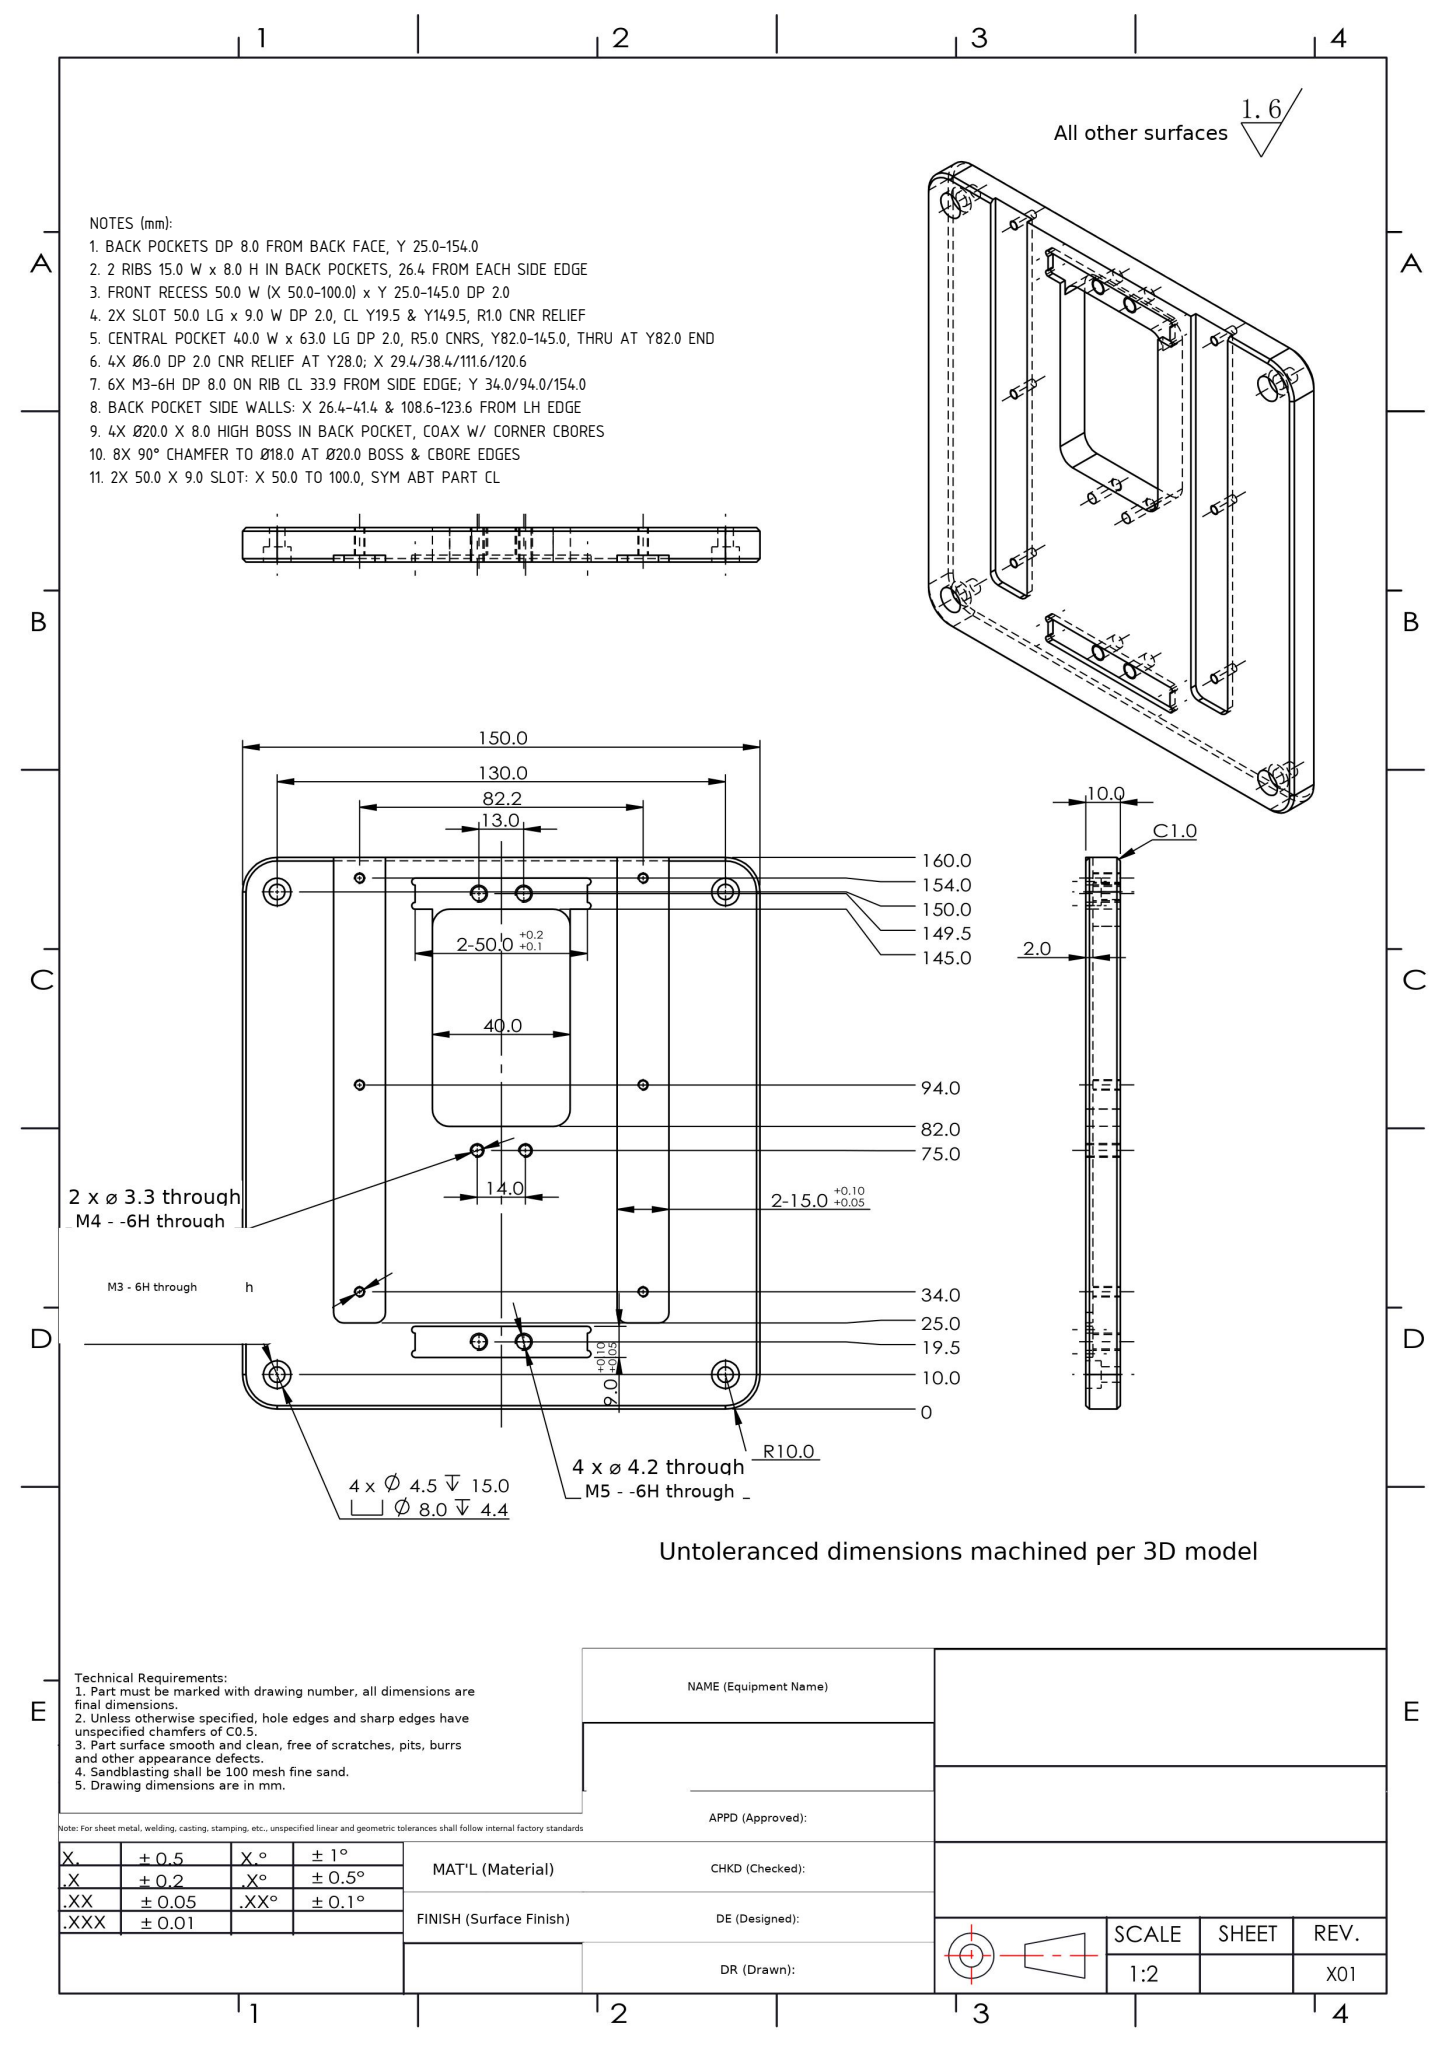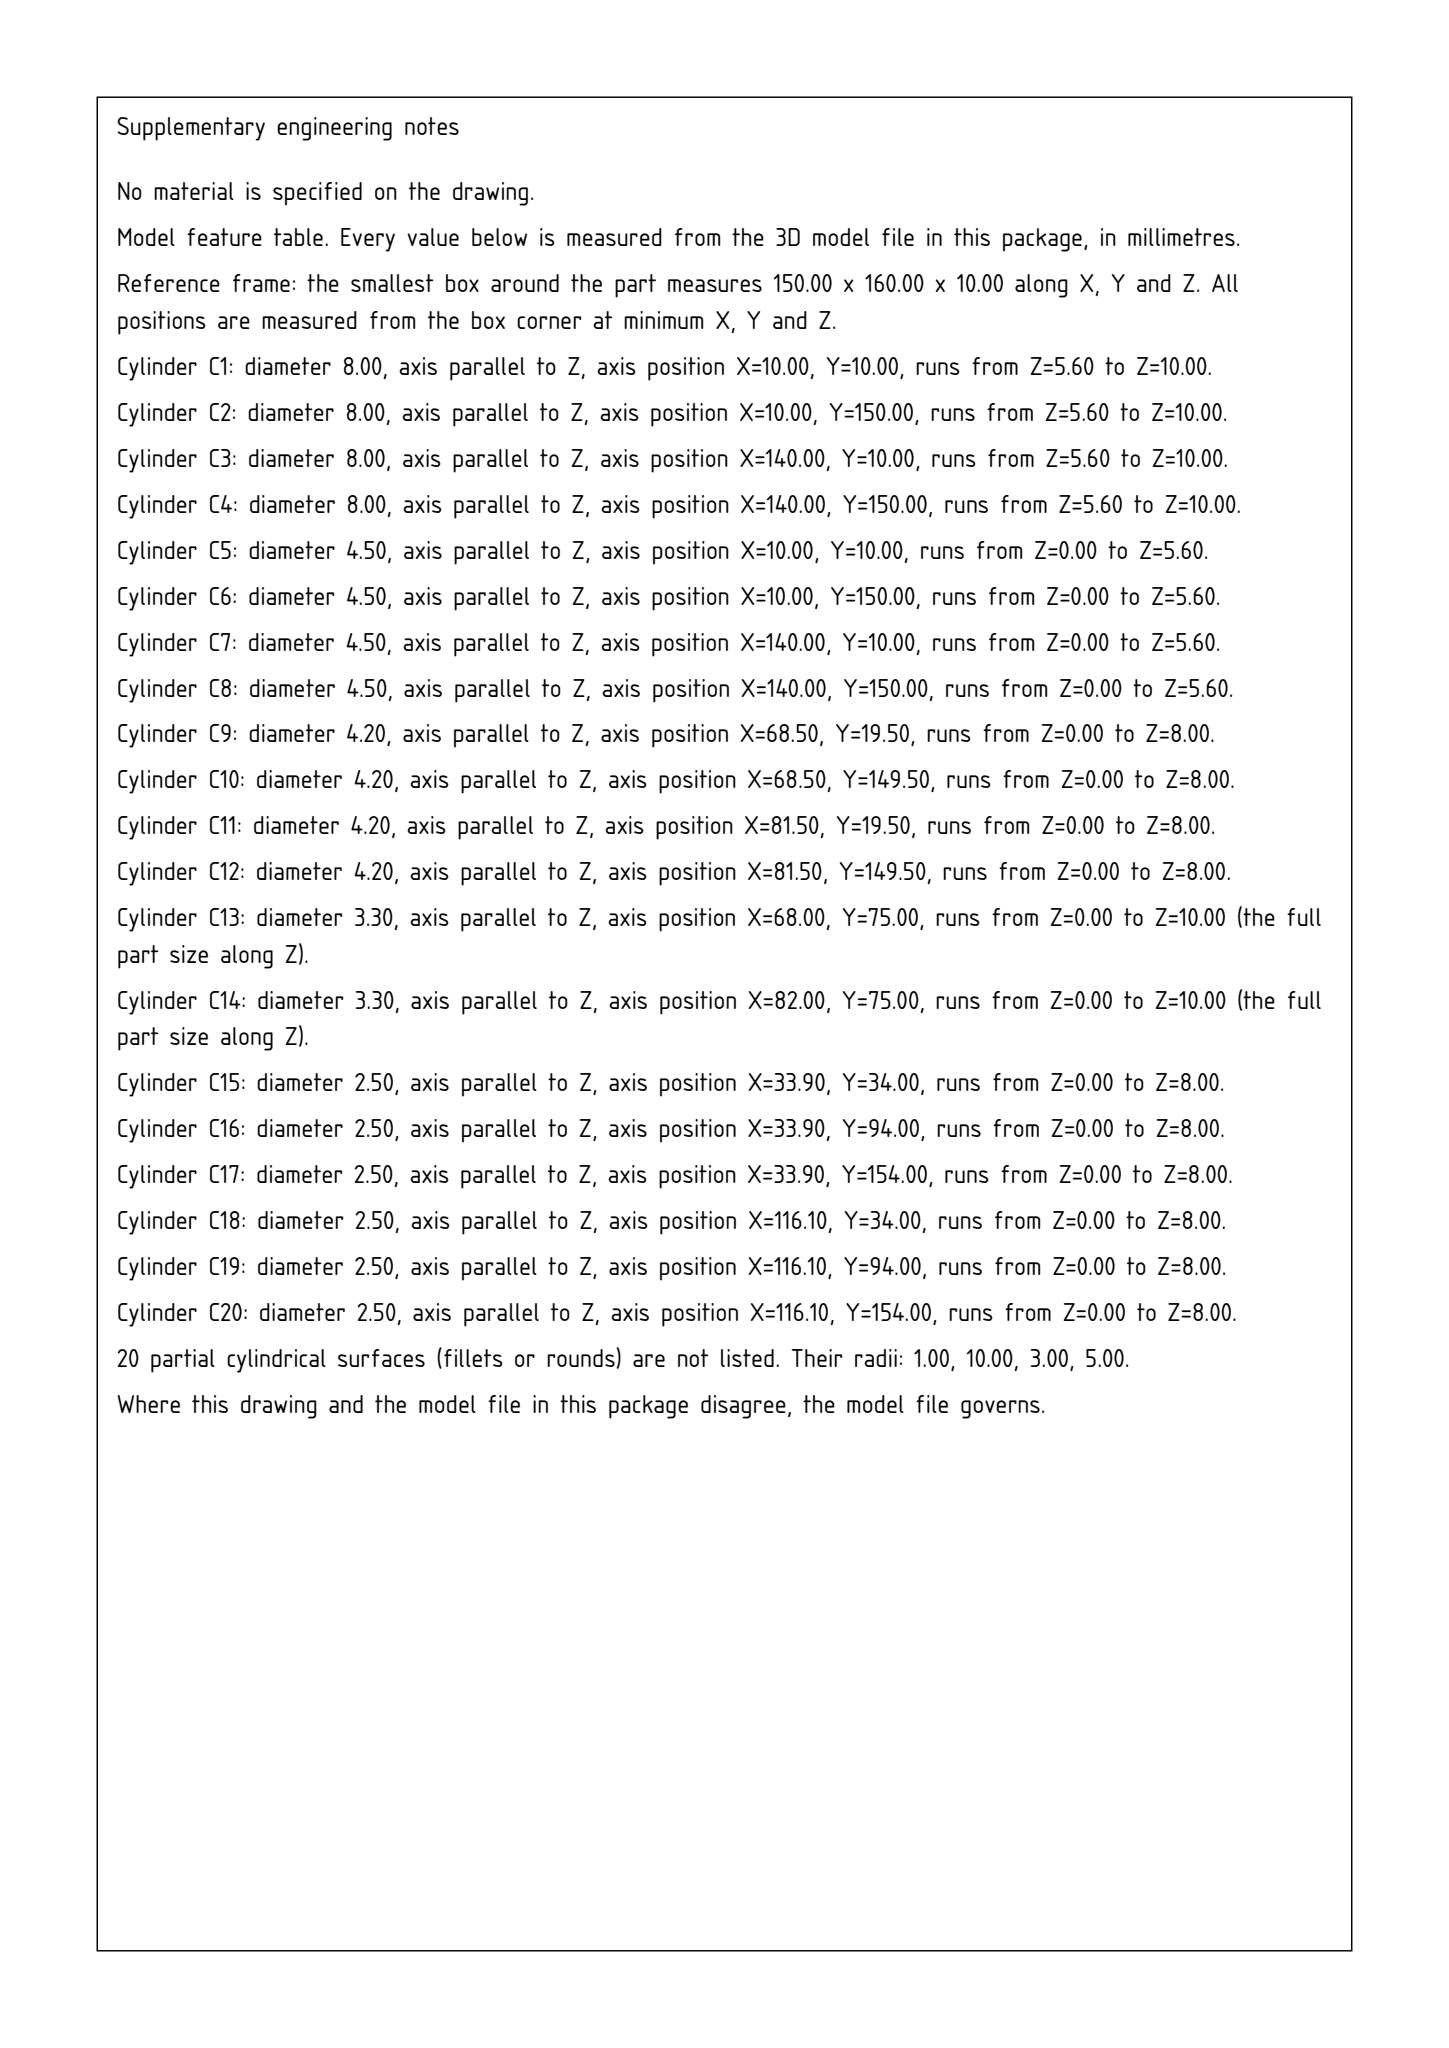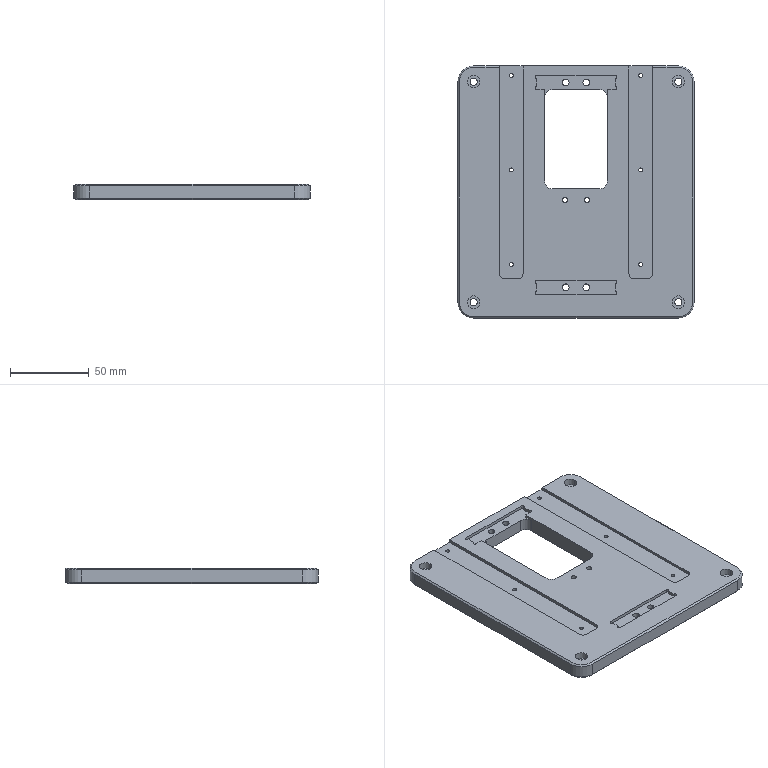Part | SolidWorks | mm | 1 solid | 114 faces | box 150 x 160 x 10 mm | volume 201582 mm3 | cylinder 64 | plane 42 | cone 8 | commonest cylinder face diameters 2 x12 2.5 x12 4.2 x8 8 x8 4.5 x8 3.3 x4 6 x4 20 x4
Drawing notes:
BACK POCKETS DP 8.0 FROM BACK FACE, Y 25.0-154.0 | from the solid: z-planes 0/8.0 (4 faces)/10.0 -> 8.0 dp pockets, 2.0 web; y-planes 25.0 (2x) and 154.0
2 RIBS 15.0 W x 8.0 H IN BACK POCKETS, 26.4 FROM EACH SIDE EDGE | from the solid: x-planes 26.4/41.4 and 108.6/123.6 = 15.0 W ribs, 26.4 from x=0 and x=150; rib top z=8.0
FRONT RECESS 50.0 W (X 50.0-100.0) x Y 25.0-145.0 DP 2.0 | from the solid: x-planes 50.0 & 100.0, y-planes 25.0 & 145.0, floor z=8.0 below front face z=10.0
2X SLOT 50.0 LG x 9.0 W DP 2.0, CL Y19.5 & Y149.5, R1.0 CNR RELIEF | from the solid: y 15.0/24.0 and 145.0/154.0 = 9.0 W, CL 19.5/149.5; x 50.0-100.0; O2.0 x 2.0 lg cyls at (50,16)(50,23)(100,16)(100,23)
CENTRAL POCKET 40.0 W x 63.0 LG DP 2.0, R5.0 CNRS, Y82.0-145.0, THRU AT Y82.0 END | from the solid: planes x55.0/95.0, y82.0/145.0; O10.0 cyls len 8.0 at (60,140)(90,140) and len 10.0 (thru) at (60,87)(90,87)
4X Ø6.0 DP 2.0 CNR RELIEF AT Y28.0; X 29.4/38.4/111.6/120.6 | from the solid: O6.0 z-cyls len 2.0 at (29.4,28),(38.4,28),(111.6,28),(120.6,28)
6X M3-6H DP 8.0 ON RIB CL 33.9 FROM SIDE EDGE; Y 34.0/94.0/154.0 | from the solid: O2.5 x 8.0 lg holes at x=33.9 & 116.1 (rib CL), y=34.0, 94.0, 154.0
BACK POCKET SIDE WALLS: X 26.4-41.4 & 108.6-123.6 FROM LH EDGE | from the solid: axis_planes x = 26.4, 41.4, 108.6, 123.6 (each 15.0 wide, CL 33.9/116.1 = M3 hole CL), pocket Y 25.0-154.0, DP 8.0 (z plane 8.0 x4)
4X Ø20.0 X 8.0 HIGH BOSS IN BACK POCKET, COAX W/ CORNER CBORES | from the solid: cylinders [20.0, z, (10,10)(10,150)(140,10)(140,150), L=8.0] coaxial with Ø4.5/Ø8.0 corner holes
8X 90° CHAMFER TO Ø18.0 AT Ø20.0 BOSS & CBORE EDGES | from the solid: cones [included_angle 90.0, ref_dia 18.0] count 8
2X 50.0 X 9.0 SLOT: X 50.0 TO 100.0, SYM ABT PART CL | from the solid: axis_planes x=50.0 (2), x=100.0 (2); y=15.0/24.0 and y=145.0/154.0 give 9.0 width at CL 19.5 & 149.5; bbox X 150.0 so CL = 75.0
build123d program:
from build123d import *

# Parameters (mm, degrees)
BOSS_EXTRUDE1_DEPTH                             = 10
CUT_EXTRUDE1_DEPTH                              = 111.114
M4_HEX_SOCKET_HEAD_CAP_SCREW_CBORE1_D           = 4.5
M4_HEX_SOCKET_HEAD_CAP_SCREW_CBORE1_DEPTH       = 15
M4_HEX_SOCKET_HEAD_CAP_SCREW_CBORE1_CBORE_D     = 8
M4_HEX_SOCKET_HEAD_CAP_SCREW_CBORE1_CBORE_DEPTH = 4.4
M4_HEX_SOCKET_HEAD_CAP_SCREW_CBORE1_TIP         = 1.352
CUT_EXTRUDE2_DEPTH                              = 2
FILLET1_R                                       = 3
M3_TAPPED_HOLE1_D                               = 2.5
FILLET2_R                                       = 10
FILLET3_R                                       = 5
SKETCH10_W                                      = 50
SKETCH10_H                                      = 9
SKETCH10_H_2                                    = 9
CUT_EXTRUDE3_DEPTH                              = 2
SKETCH11_W                                      = 5
SKETCH11_H                                      = 5
CUT_EXTRUDE4_DEPTH                              = 2
HOLE1_AT_2_COUNT                                = 2
HOLE1_AT_2_PITCH                                = 7
HOLE1_AT_3_COUNT                                = 2
HOLE1_AT_3_PITCH                                = 50.488
HOLE1_AT_4_COUNT                                = 2
HOLE1_AT_4_PITCH                                = 50
HOLE1_AT_5_COUNT                                = 2
HOLE1_AT_5_PITCH                                = 139.284
HOLE1_AT_6_COUNT                                = 2
HOLE1_AT_6_PITCH                                = 145.839
HOLE1_AT_7_COUNT                                = 2
HOLE1_AT_7_PITCH                                = 137
HOLE1_AT_8_COUNT                                = 2
HOLE1_AT_8_PITCH                                = 130
M5_TAPPED_HOLE2_D                               = 4.2
CHAMFER1_SIZE                                   = 1
M4_TAPPED_HOLE1_D                               = 3.3


with BuildPart() as part:
    # Sketch1 → Boss-Extrude1 (new body)
    with BuildSketch(Plane.XY):
        Polygon((75, -80), (-75, -80), (-75, 80), (75, 80), align=None)
    extrude(amount=BOSS_EXTRUDE1_DEPTH)

    # Sketch2 → Cut-Extrude1 (cut, through all)
    with BuildSketch(Plane(origin=(0, 0, 0), x_dir=(-1, 0, 0), z_dir=(0, 0, -1))):
        Polygon((20, 65), (-20, 65), (-20, 2), (20, 2), align=None)
    extrude(amount=-CUT_EXTRUDE1_DEPTH, mode=Mode.SUBTRACT)

    # M4 Hex Socket Head Cap Screw CBORE1
    with Locations(Plane.XY.offset(10)):
        with Locations((-65, -70), (65, -70), (65, 70), (-65, 70)):
            CounterBoreHole(M4_HEX_SOCKET_HEAD_CAP_SCREW_CBORE1_D / 2, M4_HEX_SOCKET_HEAD_CAP_SCREW_CBORE1_CBORE_D / 2, M4_HEX_SOCKET_HEAD_CAP_SCREW_CBORE1_CBORE_DEPTH, depth=M4_HEX_SOCKET_HEAD_CAP_SCREW_CBORE1_DEPTH)
            with Locations((0, 0, -(M4_HEX_SOCKET_HEAD_CAP_SCREW_CBORE1_DEPTH + M4_HEX_SOCKET_HEAD_CAP_SCREW_CBORE1_TIP / 2))):  # 118° drill point
                Cone(0, M4_HEX_SOCKET_HEAD_CAP_SCREW_CBORE1_D / 2, M4_HEX_SOCKET_HEAD_CAP_SCREW_CBORE1_TIP, mode=Mode.SUBTRACT)

    # Sketch5 → Cut-Extrude2 (cut)
    with BuildSketch(Plane.XY.offset(10)):
        Polygon((-48.6, 80), (-33.6, 80), (-33.6, -55), (-48.6, -55), align=None)
        Polygon((33.6, 80), (48.6, 80), (48.6, -55), (33.6, -55), align=None)
    extrude(amount=-CUT_EXTRUDE2_DEPTH, mode=Mode.SUBTRACT)

    # Fillet1
    fillet1_edges = [part.edges().sort_by_distance(p)[0] for p in [
        (-48.6, -55, 9),
        (-33.6, -55, 9),
        (33.6, -55, 9),
        (48.6, -55, 9),
    ]]
    fillet(fillet1_edges, radius=FILLET1_R)

    # M3 Tapped Hole1 (through all)
    with Locations(Plane.XY.offset(10)):
        with Locations((41.1, 74), (41.1, 14), (41.1, -46), (-41.1, -46), (-41.1, 14), (-41.1, 74)):
            Hole(M3_TAPPED_HOLE1_D / 2)

    # Fillet2
    fillet2_edges = [part.edges().sort_by_distance(p)[0] for p in [
        (-75, 80, 5),
        (75, 80, 5),
        (75, -80, 5),
        (-75, -80, 5),
    ]]
    fillet(fillet2_edges, radius=FILLET2_R)

    # Fillet3
    fillet3_edges = [part.edges().sort_by_distance(p)[0] for p in [
        (20, 2, 5),
        (20, 65, 5),
        (-20, 65, 5),
        (-20, 2, 5),
    ]]
    fillet(fillet3_edges, radius=FILLET3_R)

    # Sketch10 → Cut-Extrude3 (cut)
    with BuildSketch(Plane(origin=(0, 0, 10), x_dir=(-1, 0, 0), z_dir=(0, 0, -1))):
        with Locations((0, 69.5)):
            Rectangle(SKETCH10_W, SKETCH10_H)
        with Locations((0, -60.5)):
            Rectangle(SKETCH10_W, SKETCH10_H_2)
    extrude(amount=CUT_EXTRUDE3_DEPTH, mode=Mode.SUBTRACT)

    # Sketch11 → Cut-Extrude4 (cut)
    with BuildSketch(Plane(origin=(0, 0, 10), x_dir=(-1, 0, 0), z_dir=(0, 0, -1))):
        with Locations((-17.5, 62.5)):
            Rectangle(SKETCH11_W, SKETCH11_H)
        with Locations((17.5, 62.5)):
            Rectangle(SKETCH11_W, SKETCH11_H)
    extrude(amount=CUT_EXTRUDE4_DEPTH, mode=Mode.SUBTRACT)

    # Sketch12 → Hole1 (revolve, cut)
    with BuildSketch(Plane(origin=(-25, 73, 10), x_dir=(0, -1, 0), z_dir=(1, 0, 0))):
        Polygon((0, 0), (0, 1.999), (1, 1.999), (1, 0), align=None)
    hole1 = revolve(axis=Axis((-25, 73, 10), (0, 0, -1)), mode=Mode.SUBTRACT)

    # Hole1 at 2: Hole1 ×2
    with Locations(*[(0, -i * HOLE1_AT_2_PITCH, 0) for i in range(1, HOLE1_AT_2_COUNT)]):
        add(hole1, mode=Mode.SUBTRACT)

    # Hole1 at 3: Hole1 ×2
    with Locations(*[Vector(0.9903, -0.1386, 0) * (i * HOLE1_AT_3_PITCH) for i in range(1, HOLE1_AT_3_COUNT)]):
        add(hole1, mode=Mode.SUBTRACT)

    # Hole1 at 4: Hole1 ×2
    with Locations(*[(i * HOLE1_AT_4_PITCH, 0, 0) for i in range(1, HOLE1_AT_4_COUNT)]):
        add(hole1, mode=Mode.SUBTRACT)

    # Hole1 at 5: Hole1 ×2
    with Locations(*[Vector(0.359, -0.9333, 0) * (i * HOLE1_AT_5_PITCH) for i in range(1, HOLE1_AT_5_COUNT)]):
        add(hole1, mode=Mode.SUBTRACT)

    # Hole1 at 6: Hole1 ×2
    with Locations(*[Vector(0.3428, -0.9394, 0) * (i * HOLE1_AT_6_PITCH) for i in range(1, HOLE1_AT_6_COUNT)]):
        add(hole1, mode=Mode.SUBTRACT)

    # Hole1 at 7: Hole1 ×2
    with Locations(*[(0, -i * HOLE1_AT_7_PITCH, 0) for i in range(1, HOLE1_AT_7_COUNT)]):
        add(hole1, mode=Mode.SUBTRACT)

    # Hole1 at 8: Hole1 ×2
    with Locations(*[(0, -i * HOLE1_AT_8_PITCH, 0) for i in range(1, HOLE1_AT_8_COUNT)]):
        add(hole1, mode=Mode.SUBTRACT)

    # M5 Tapped Hole2 (through all)
    with Locations(Plane.XY.offset(8)):
        with Locations((6.5, -60.5), (-6.5, -60.5), (6.5, 69.5), (-6.5, 69.5)):
            Hole(M5_TAPPED_HOLE2_D / 2)

    # Chamfer1
    chamfer1_edges = [part.edges().sort_by_distance(p)[0] for p in [
        (-75, 0, 0),
        (-75, 0, 10),
        (0, 80, 0),
        (75, 0, 0),
        (0, -80, 0),
        (-72.071, -77.071, 0),
        (72.071, -77.071, 0),
        (72.071, 77.071, 0),
        (-72.071, 77.071, 0),
        (56.8, 80, 10),
        (0, -80, 10),
        (75, 0, 10),
        (-72.071, -77.071, 10),
        (72.071, -77.071, 10),
        (72.071, 77.071, 10),
        (-72.071, 77.071, 10),
        (-56.8, 80, 10),
    ]]
    chamfer(chamfer1_edges, length=CHAMFER1_SIZE)

    # M4 Tapped Hole1 (through all)
    with Locations(Plane(origin=(0, 0, 0), x_dir=(-1, 0, 0), z_dir=(0, 0, -1))):
        with Locations((-7, -5), (7, -5)):
            Hole(M4_TAPPED_HOLE1_D / 2)


solid = part.part